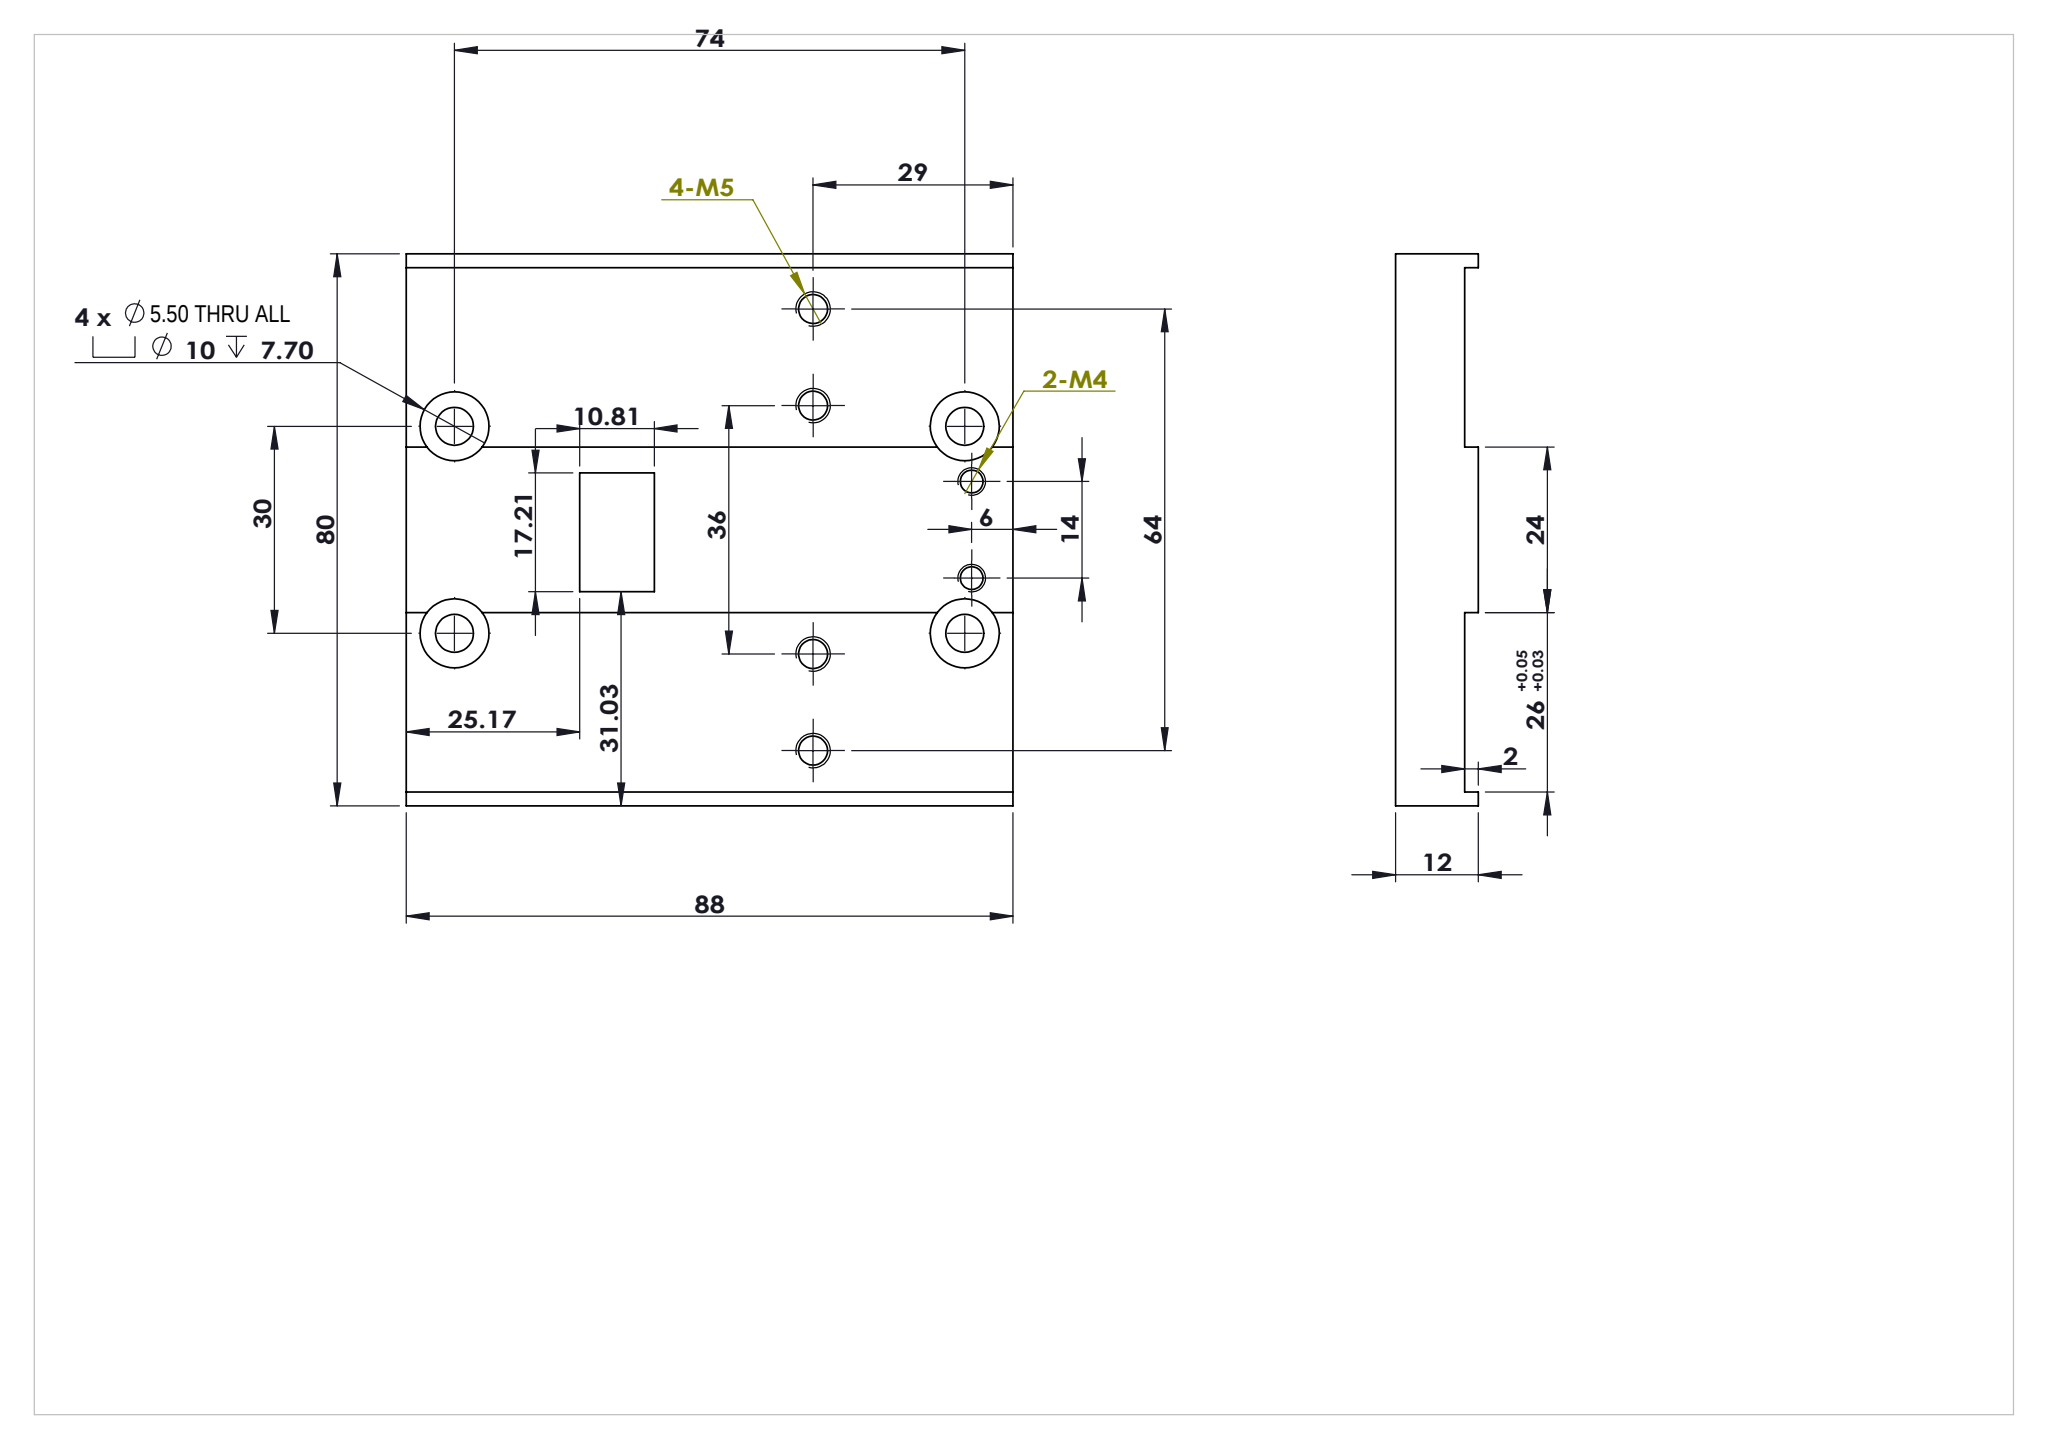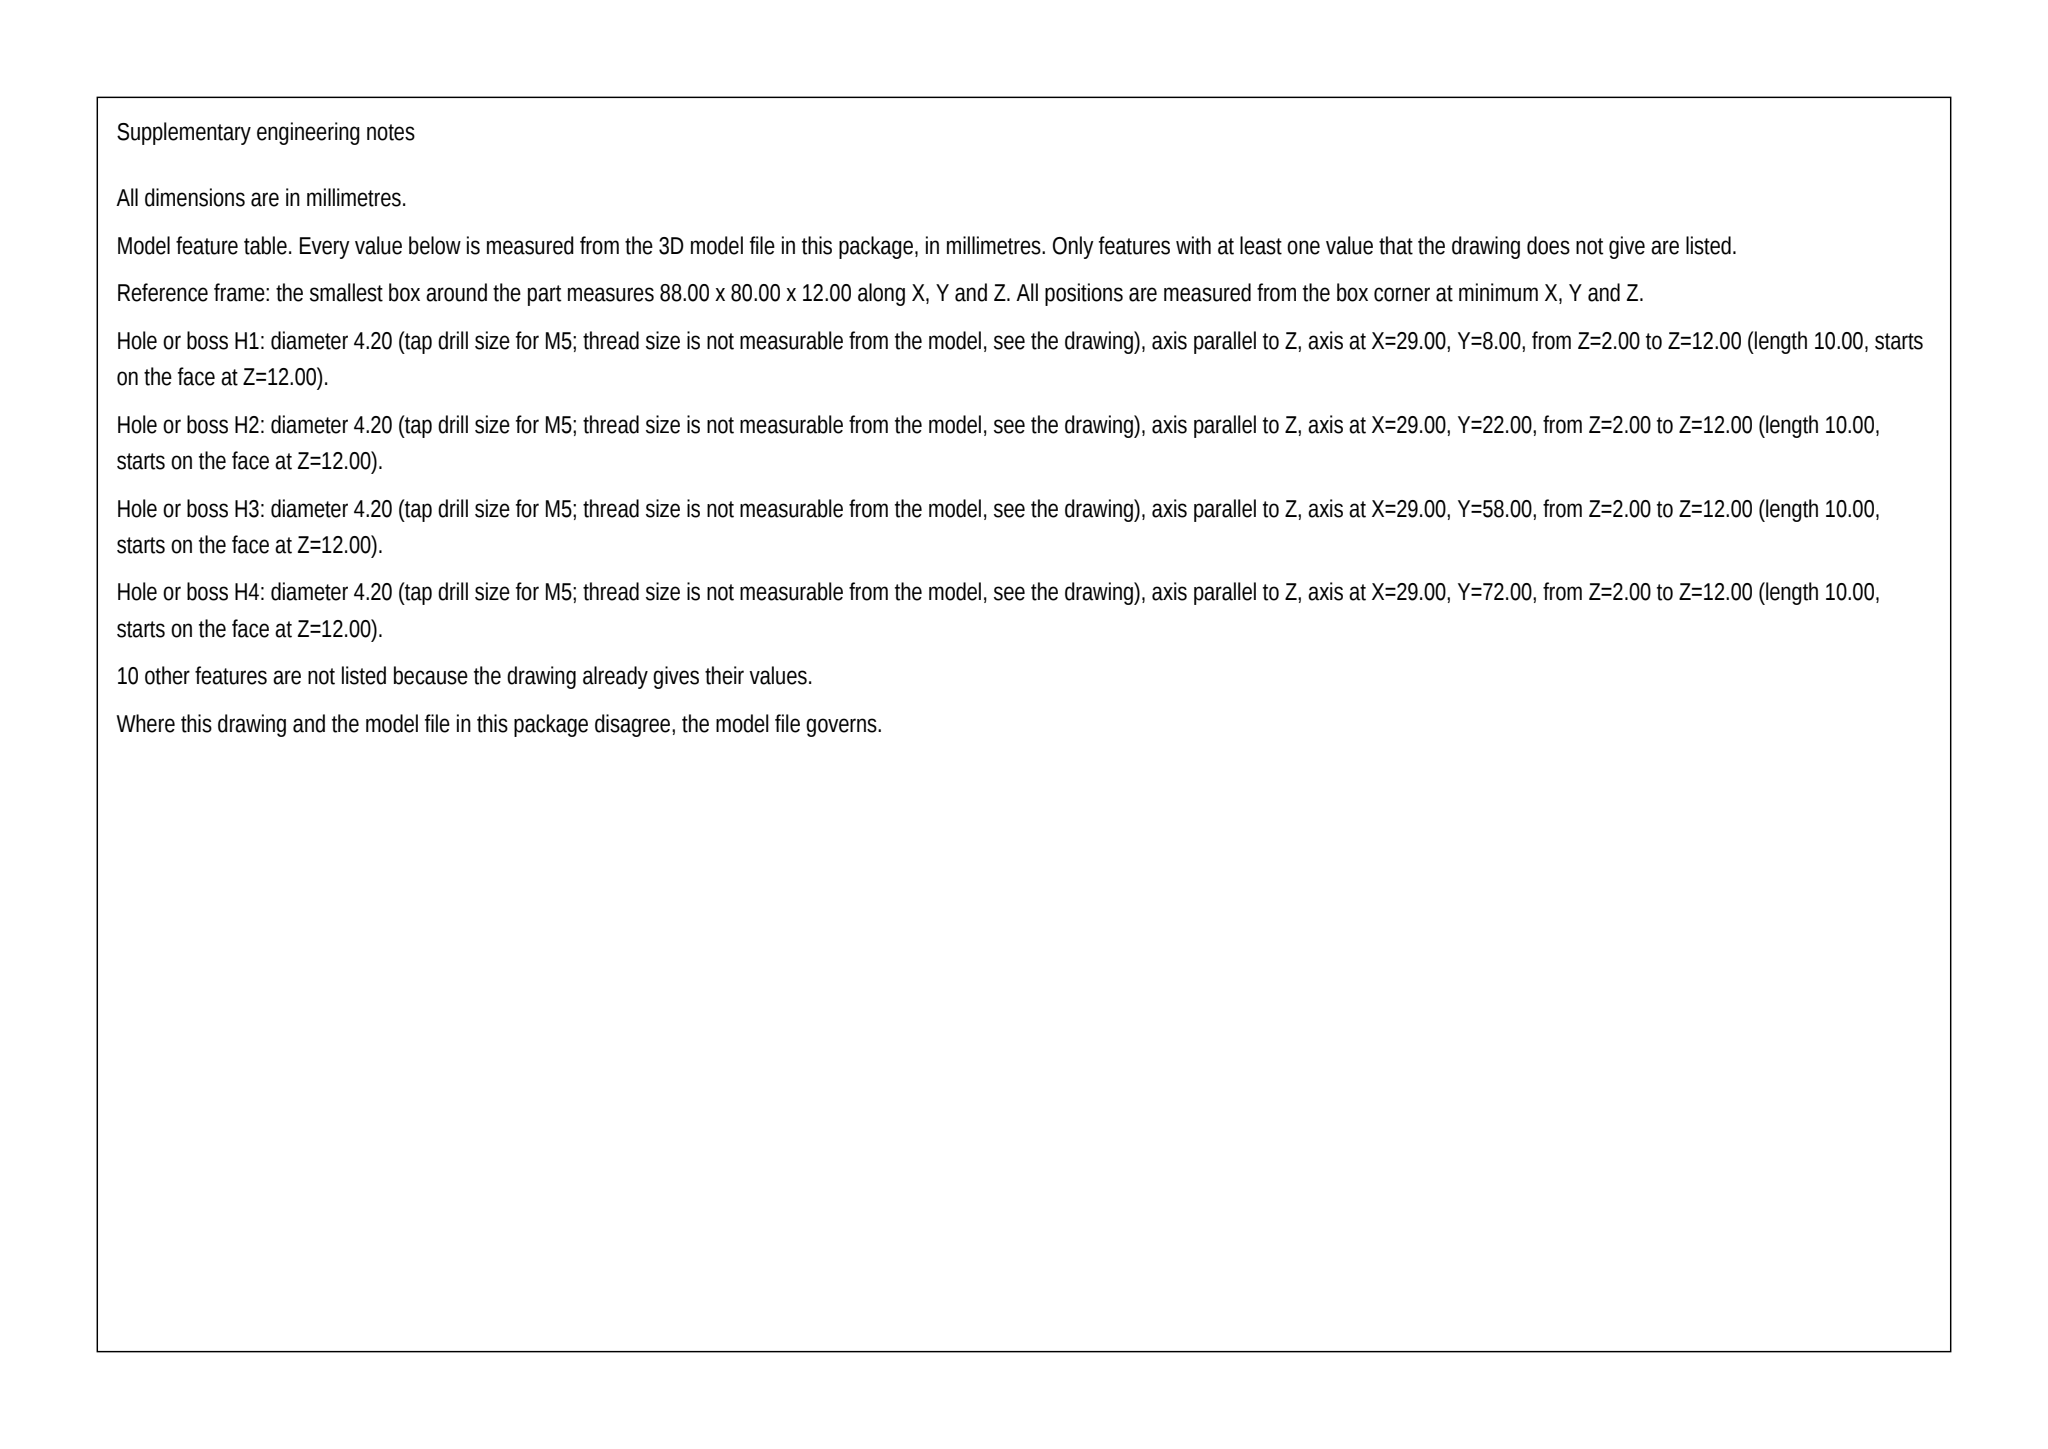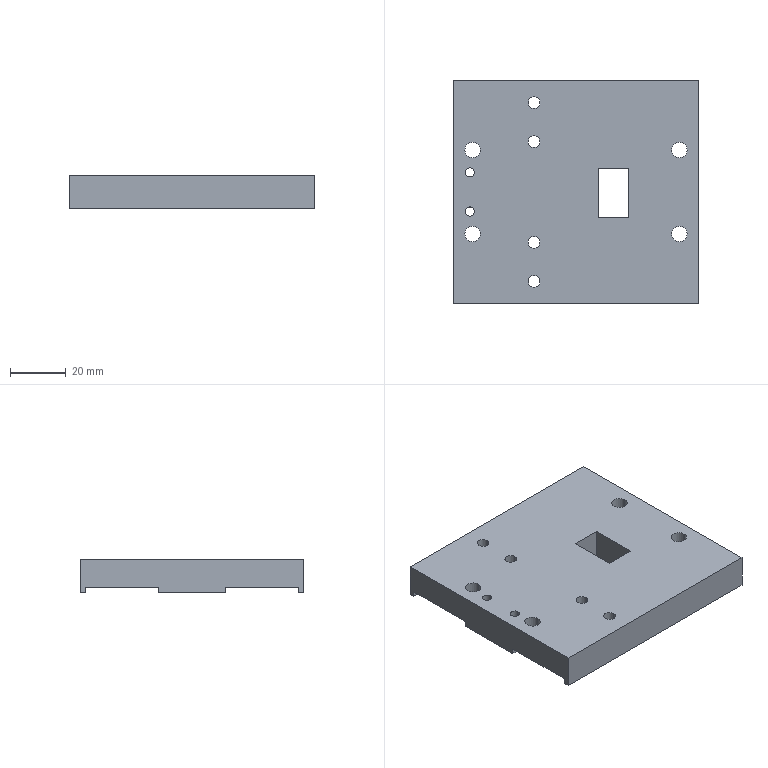Part | SolidWorks | mm | 1 solid | 54 faces | box 88 x 80 x 12 mm | volume 70046 mm3 | cylinder 28 | plane 26 | commonest cylinder face diameters 4.2 x8 10 x8 5.5 x8 3.3 x4
build123d program:
from build123d import *

# Parameters (mm, degrees)
SKETCH1_W                                            = 88
SKETCH1_H                                            = 80
BOSS_EXTRUDE1_DEPTH                                  = 12
HOLE_SIZE_ACCORDING_TO_THE_TYPE_OF_HEX_S_D           = 5.5
HOLE_SIZE_ACCORDING_TO_THE_TYPE_OF_HEX_S_CBORE_D     = 10
HOLE_SIZE_ACCORDING_TO_THE_TYPE_OF_HEX_S_CBORE_DEPTH = 7.7
SKETCH3_2_W                                          = 88
SKETCH3_2_H                                          = 26
CUT_EXTRUDE1_DEPTH                                   = 2
M5_TAPPED_HOLE1_D                                    = 4.2
M4_TAPPED_HOLE1_D                                    = 3.3
HOLE_SIZE_ACCORDING_TO_THE_TYPE_OF_H_2_D             = 5.5
HOLE_SIZE_ACCORDING_TO_THE_TYPE_OF_H_2_CBORE_D       = 10
HOLE_SIZE_ACCORDING_TO_THE_TYPE_OF_H_2_CBORE_DEPTH   = 5.7
SKETCH8_W                                            = 10.813
SKETCH8_H                                            = 17.211
CUT_EXTRUDE2_DEPTH                                   = 46


with BuildPart() as part:
    # Sketch1 → Boss-Extrude1 (new body)
    with BuildSketch(Plane.XY):
        Rectangle(SKETCH1_W, SKETCH1_H)
    extrude(amount=BOSS_EXTRUDE1_DEPTH)

    # Hole Size according to the type of hex s (through all)
    with Locations(Plane(origin=(0, 0, 0), x_dir=(-1, 0, 0), z_dir=(0, 0, -1))):
        with Locations((-37, 15), (-37, -15), (37, -15), (37, 15)):
            CounterBoreHole(HOLE_SIZE_ACCORDING_TO_THE_TYPE_OF_HEX_S_D / 2, HOLE_SIZE_ACCORDING_TO_THE_TYPE_OF_HEX_S_CBORE_D / 2, HOLE_SIZE_ACCORDING_TO_THE_TYPE_OF_HEX_S_CBORE_DEPTH)

    # Sketch3_2 → Cut-Extrude1 (cut)
    with BuildSketch(Plane(origin=(0, 0, 0), x_dir=(-1, 0, 0), z_dir=(0, 0, -1))):
        with Locations((0, 25)):
            Rectangle(SKETCH3_2_W, SKETCH3_2_H)
        with Locations((0, -25)):
            Rectangle(SKETCH3_2_W, SKETCH3_2_H)
    extrude(amount=-CUT_EXTRUDE1_DEPTH, mode=Mode.SUBTRACT)

    # M5 Tapped Hole1 (through all)
    with Locations(Plane(origin=(0, 0, 2), x_dir=(-1, 0, 0), z_dir=(0, 0, -1))):
        with Locations((15, -32), (15, -18)):
            m5_tapped_hole1 = Hole(M5_TAPPED_HOLE1_D / 2)

    # Mirror1: M5 Tapped Hole1 across plane
    add(m5_tapped_hole1.mirror(Plane.ZX), mode=Mode.SUBTRACT)

    # M4 Tapped Hole1 (through all)
    with Locations(Plane(origin=(0, 0, 0), x_dir=(-1, 0, 0), z_dir=(0, 0, -1))):
        with Locations((38, 7), (38, -7)):
            Hole(M4_TAPPED_HOLE1_D / 2)

    # Hole Size according to the type of h 2 (through all)
    with Locations(Plane(origin=(0, 0, 0), x_dir=(-1, 0, 0), z_dir=(0, 0, -1))):
        with Locations((-37, -15), (-37, 15), (37, -15), (37, 15)):
            CounterBoreHole(HOLE_SIZE_ACCORDING_TO_THE_TYPE_OF_H_2_D / 2, HOLE_SIZE_ACCORDING_TO_THE_TYPE_OF_H_2_CBORE_D / 2, HOLE_SIZE_ACCORDING_TO_THE_TYPE_OF_H_2_CBORE_DEPTH)

    # Sketch8 → Cut-Extrude2 (cut)
    with BuildSketch(Plane(origin=(0, 0, 0), x_dir=(-1, 0, 0), z_dir=(0, 0, -1))):
        with Locations((-13.427, -0.3604)):
            Rectangle(SKETCH8_W, SKETCH8_H)
    extrude(amount=-CUT_EXTRUDE2_DEPTH, mode=Mode.SUBTRACT)


solid = part.part